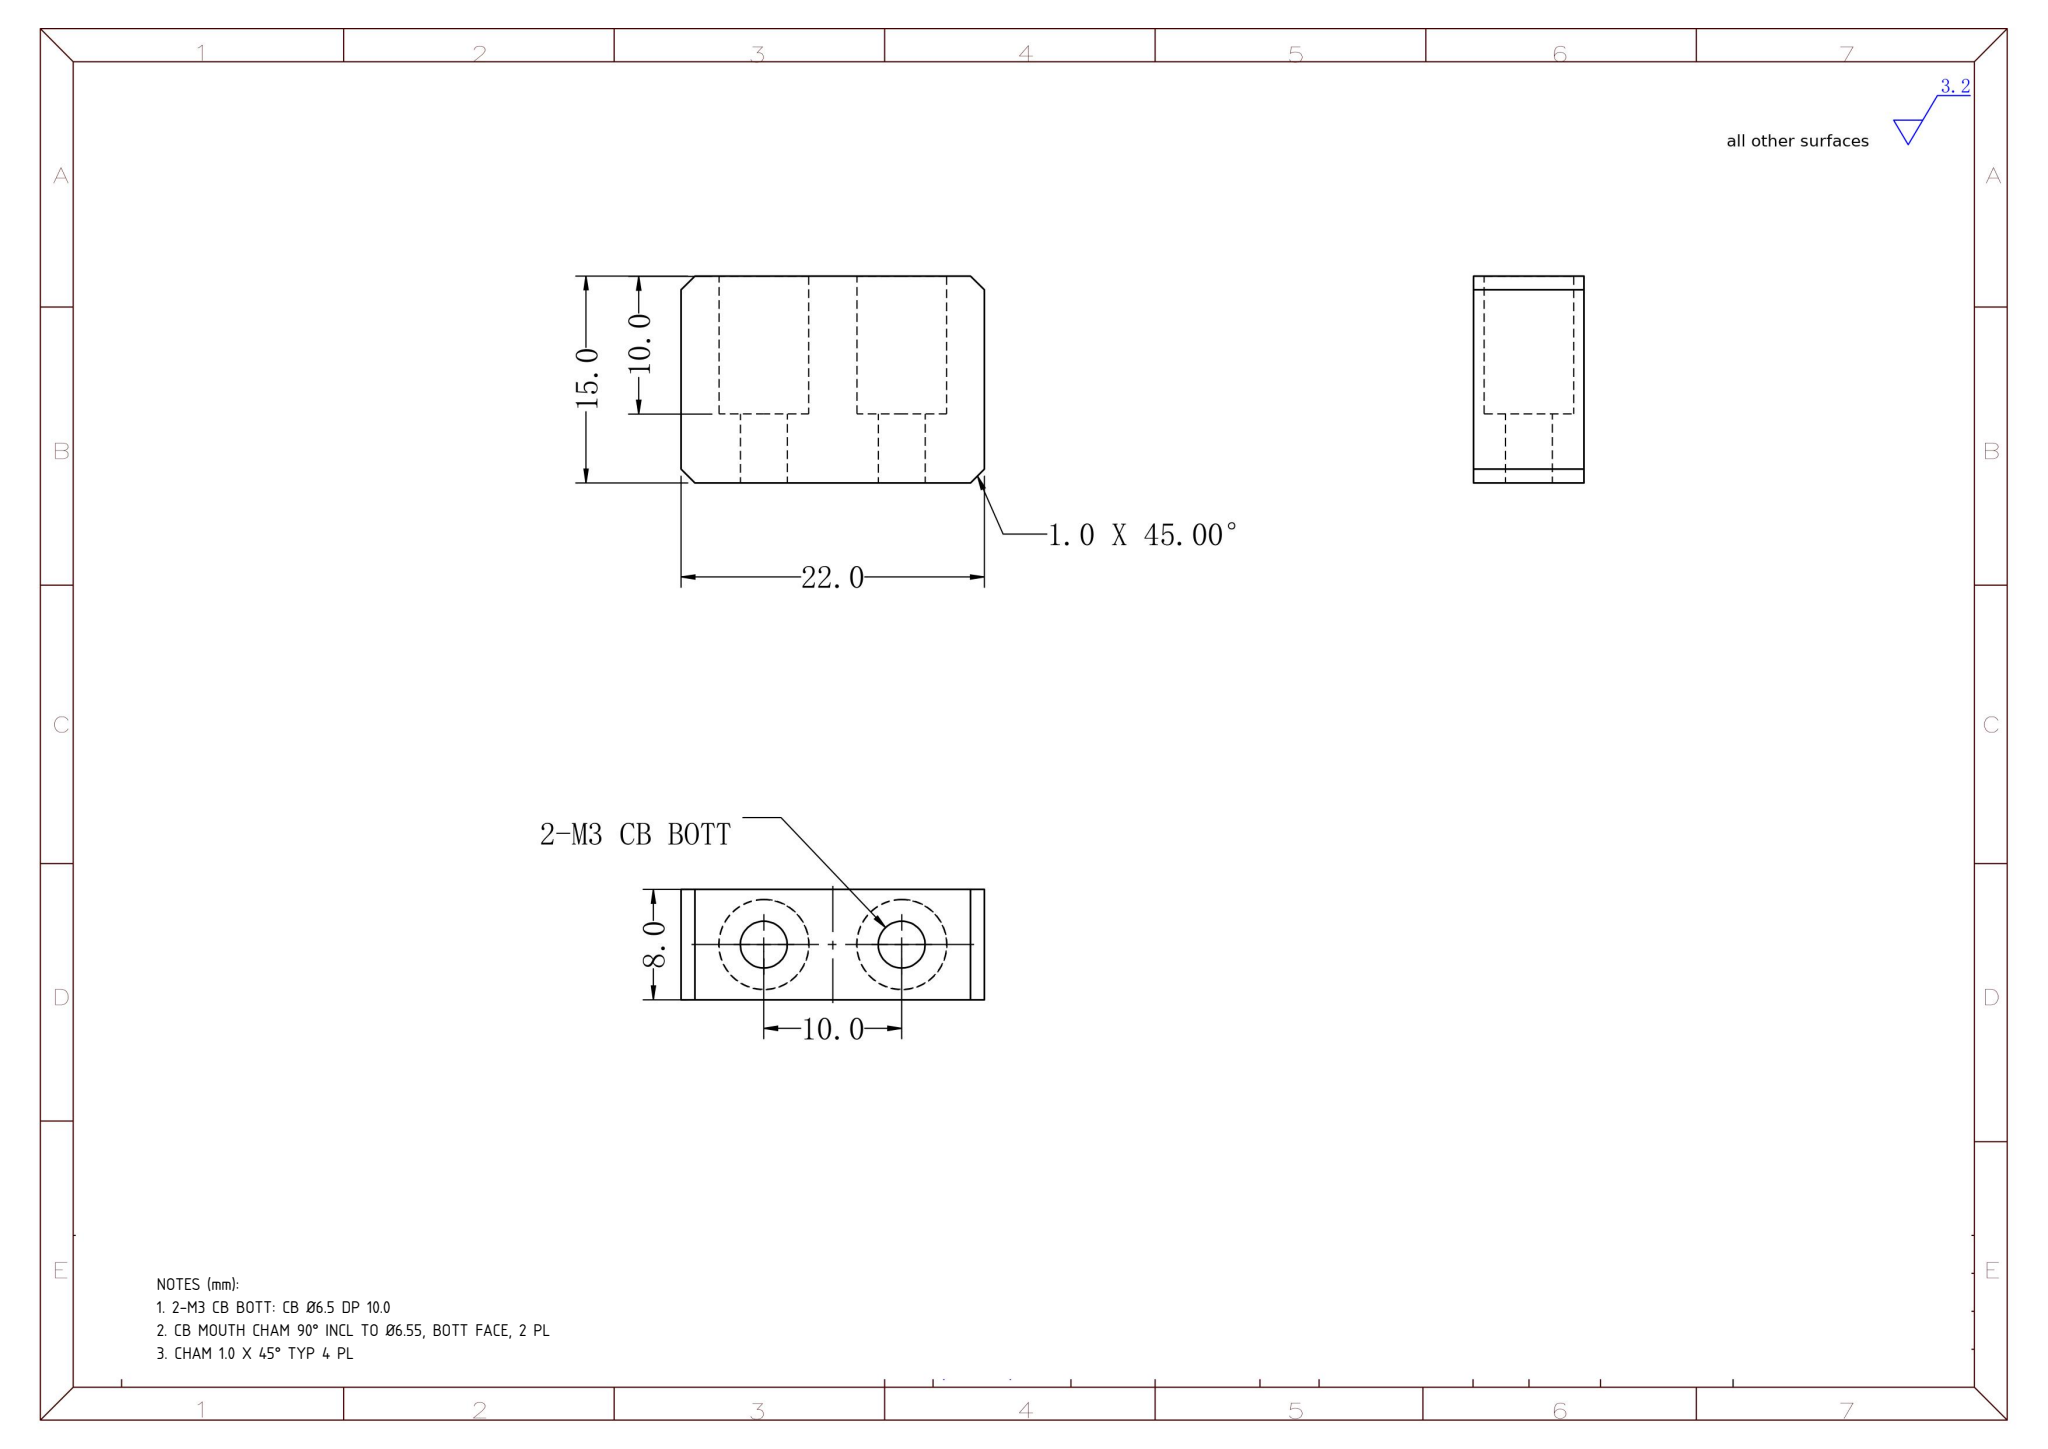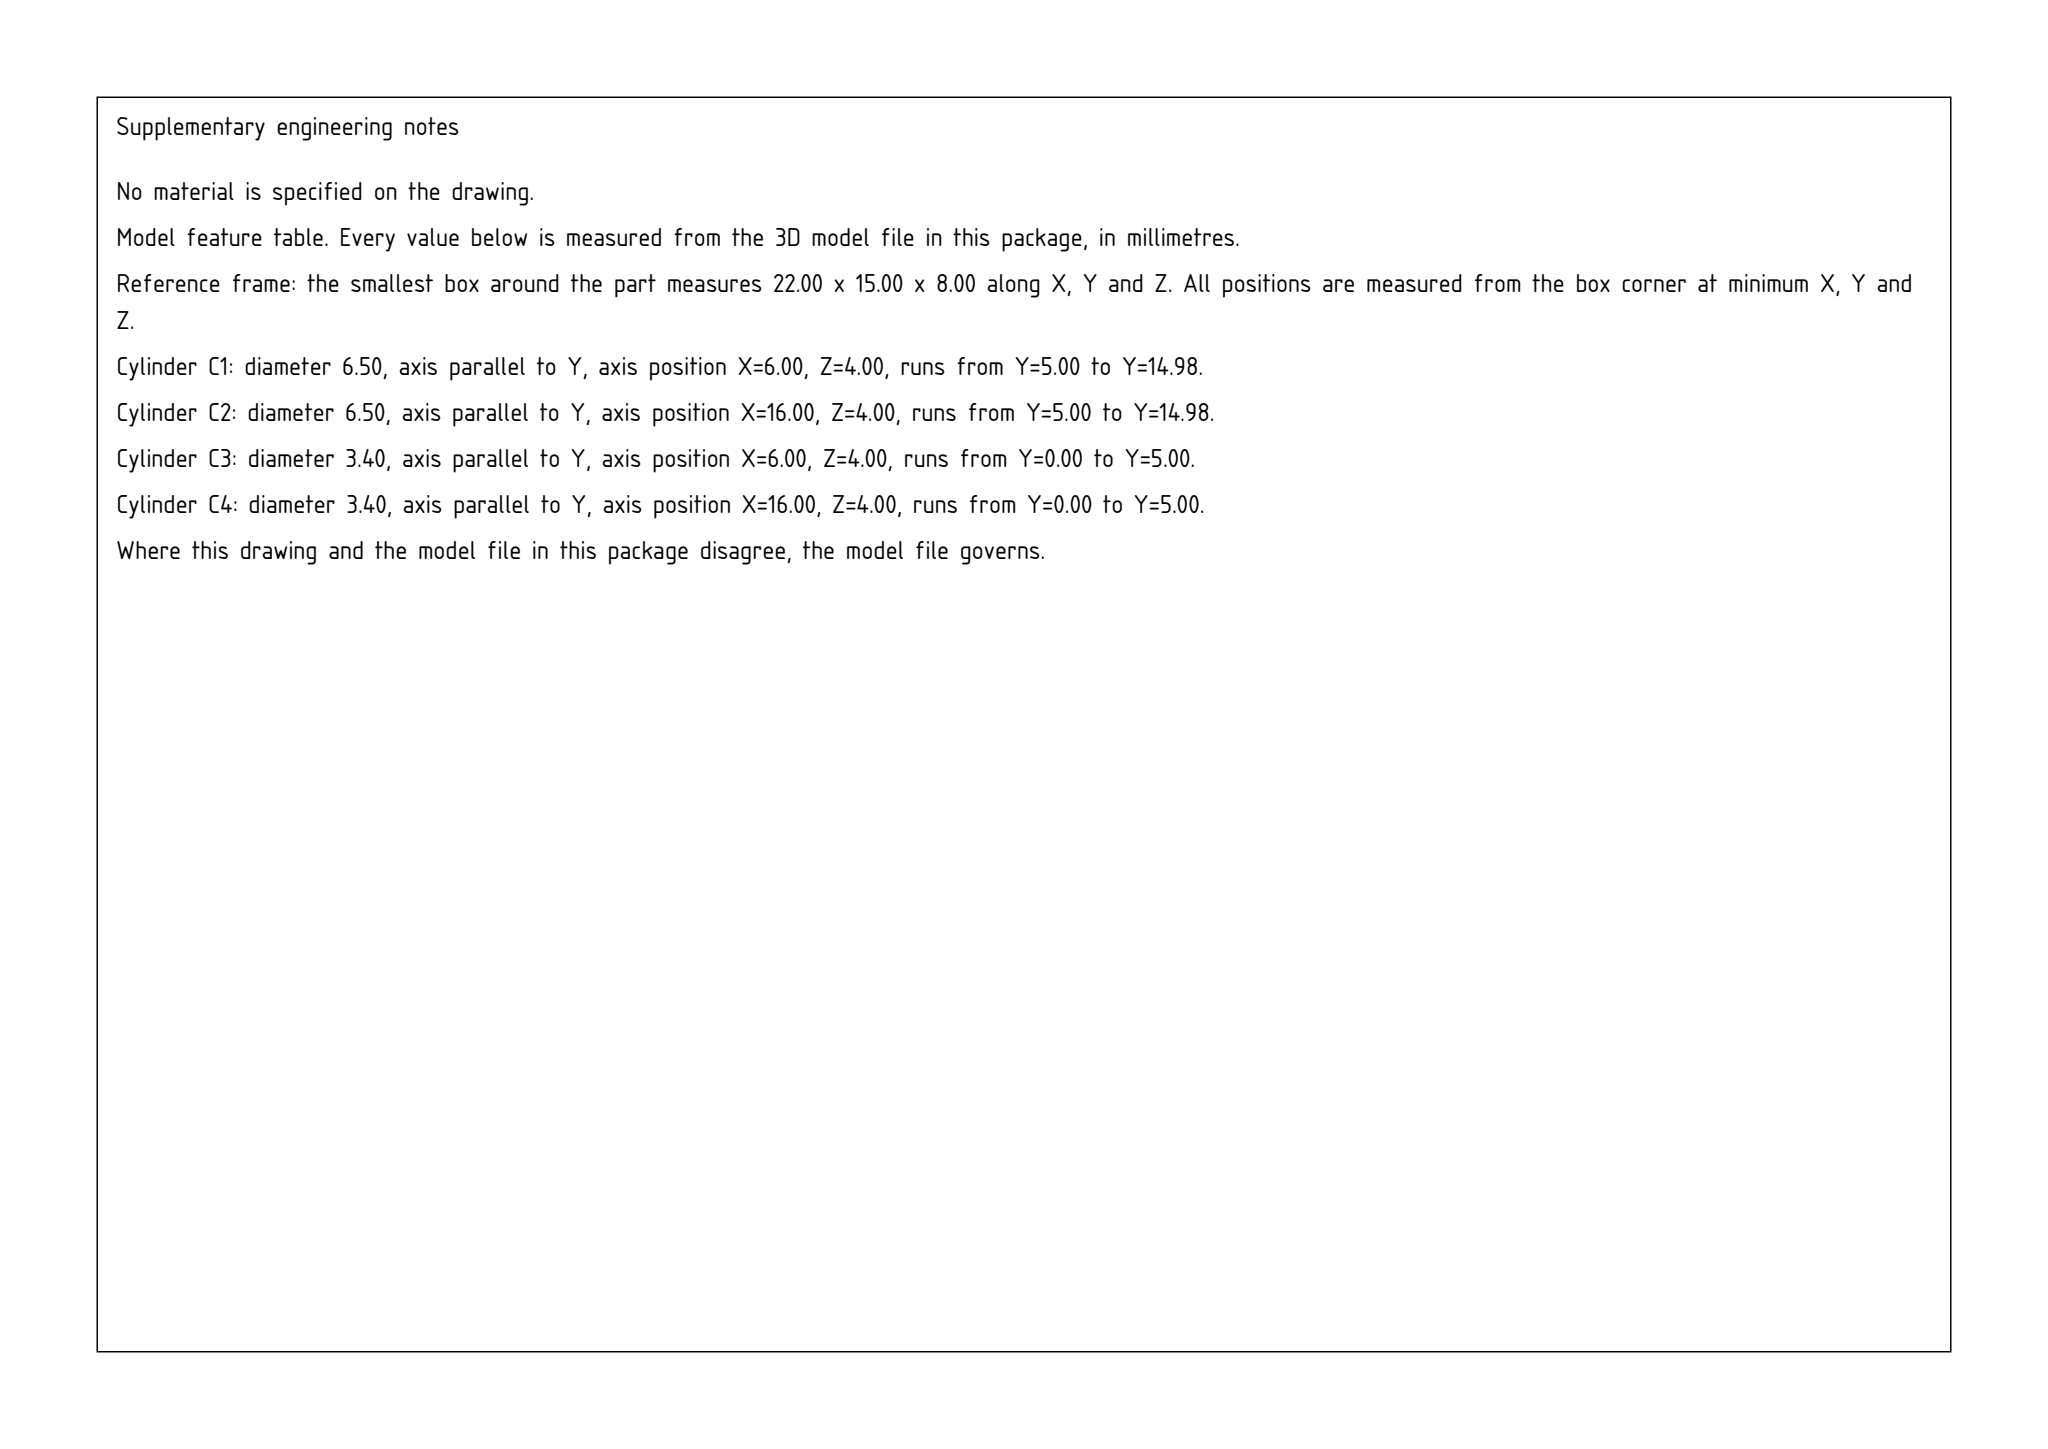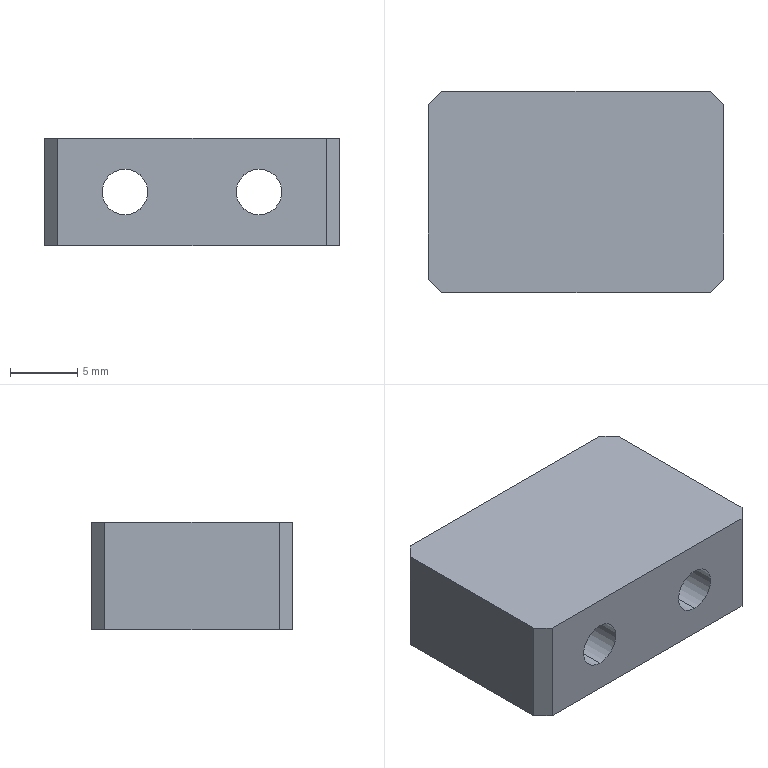Part | SolidWorks | mm | 1 solid | 24 faces | box 22 x 15 x 8 mm | volume 1870 mm3 | plane 12 | cylinder 8 | cone 4 | commonest cylinder face diameters 6.5 x4 3.4 x4
Drawing notes:
2-M3 CB BOTT: CB Ø6.5 DP 10.0 | from the solid: cylinders dia 6.5, axis y, at x=6.0 & 16.0, z=4.0, length 9.98 (y=5 to 15); matches 10.0 dim
CB MOUTH CHAM 90° INCL TO Ø6.55, BOTT FACE, 2 PL | from the solid: cones[included_angle 90.0, ref_dia 6.55] at Ø6.5 CB ends
CHAM 1.0 X 45° TYP 4 PL | from the solid: 4 corner chamfers on 22.0 x 15.0 outline, x-planes 0/22, y-planes 0/15
build123d program:
from build123d import *

# Parameters (mm, degrees)
SKETCH1_W                                      = 22
SKETCH1_H                                      = 15
BOSS_EXTRUDE1_DEPTH                            = 8
CHAMFER1_SIZE                                  = 1
M3_HEX_SOCKET_HEAD_CAP_SCREW_CBORE1_AT_2_COUNT = 2
M3_HEX_SOCKET_HEAD_CAP_SCREW_CBORE1_AT_2_PITCH = 10


with BuildPart() as part:
    # Sketch1 → Boss-Extrude1 (new body)
    with BuildSketch(Plane.XY):
        Rectangle(SKETCH1_W, SKETCH1_H)
    extrude(amount=BOSS_EXTRUDE1_DEPTH)

    # Chamfer1
    chamfer1_edges = [part.edges().sort_by_distance(p)[0] for p in [
        (11, -7.5, 4),
        (-11, -7.5, 4),
        (-11, 7.5, 4),
        (11, 7.5, 4),
    ]]
    chamfer(chamfer1_edges, length=CHAMFER1_SIZE)

    # Sketch7 → M3 Hex Socket Head Cap Screw CBORE1 (revolve, cut)
    with BuildSketch(Plane(origin=(-5, 7.5, 4), x_dir=(0, 0, 1), z_dir=(1, 0, 0))):
        Polygon((0, 0), (0, 15), (1.7, 15), (1.7, 10), (3.25, 10), (3.25, 0.025), (3.275, 0), align=None)
    m3_hex_socket_head_cap_screw_cbore1 = revolve(axis=Axis((-5, 13.85, 4), (0, -1, 0)), mode=Mode.SUBTRACT)

    # M3 Hex Socket Head Cap Screw CBORE1 at 2: M3 Hex Socket Head Cap Screw CBORE1 ×2
    with Locations(*[(i * M3_HEX_SOCKET_HEAD_CAP_SCREW_CBORE1_AT_2_PITCH, 0, 0) for i in range(1, M3_HEX_SOCKET_HEAD_CAP_SCREW_CBORE1_AT_2_COUNT)]):
        add(m3_hex_socket_head_cap_screw_cbore1, mode=Mode.SUBTRACT)


solid = part.part
STEP:
#1=CARTESIAN_POINT('',(-5.,7.475,0.75));
#2=VERTEX_POINT('',#1);
#3=CARTESIAN_POINT('',(-5.,7.475,7.25));
#4=VERTEX_POINT('',#3);
#5=CARTESIAN_POINT('',(-5.,7.475,4.));
#6=DIRECTION('',(0.,1.,0.));
#7=DIRECTION('',(0.,0.,1.));
#8=AXIS2_PLACEMENT_3D('',#5,#6,#7);
#9=CIRCLE('',#8,3.25);
#10=EDGE_CURVE('',#2,#4,#9,.T.);
#11=ORIENTED_EDGE('',*,*,#10,.F.);
#12=CARTESIAN_POINT('',(-5.,7.5,0.725));
#13=VERTEX_POINT('',#12);
#14=CARTESIAN_POINT('',(-5.,7.5,0.725));
#15=DIRECTION('',(0.,0.7071,-0.7071));
#16=VECTOR('',#15,1000.);
#17=LINE('',#14,#16);
#18=EDGE_CURVE('',#2,#13,#17,.T.);
#19=ORIENTED_EDGE('',*,*,#18,.T.);
#20=CARTESIAN_POINT('',(-5.,7.5,7.275));
#21=VERTEX_POINT('',#20);
#22=CARTESIAN_POINT('',(-5.,7.5,4.));
#23=DIRECTION('',(0.,1.,0.));
#24=DIRECTION('',(0.,0.,1.));
#25=AXIS2_PLACEMENT_3D('',#22,#23,#24);
#26=CIRCLE('',#25,3.275);
#27=EDGE_CURVE('',#13,#21,#26,.T.);
#28=ORIENTED_EDGE('',*,*,#27,.T.);
#29=CARTESIAN_POINT('',(-5.,7.5,7.275));
#30=DIRECTION('',(0.,0.7071,0.7071));
#31=VECTOR('',#30,1000.);
#32=LINE('',#29,#31);
#33=EDGE_CURVE('',#4,#21,#32,.T.);
#34=ORIENTED_EDGE('',*,*,#33,.F.);
#35=EDGE_LOOP('',(#11,#19,#28,#34));
#36=FACE_OUTER_BOUND('',#35,.T.);
#37=CARTESIAN_POINT('',(-5.,7.5,4.));
#38=DIRECTION('',(0.,1.,0.));
#39=DIRECTION('',(0.,0.,1.));
#40=AXIS2_PLACEMENT_3D('',#37,#38,#39);
#41=CONICAL_SURFACE('',#40,3.275,0.7854);
#42=ADVANCED_FACE('',(#36),#41,.F.);
#43=CARTESIAN_POINT('',(-5.,-2.5,0.75));
#44=VERTEX_POINT('',#43);
#45=CARTESIAN_POINT('',(-5.,-2.5,7.25));
#46=VERTEX_POINT('',#45);
#47=CARTESIAN_POINT('',(-5.,-2.5,4.));
#48=DIRECTION('',(0.,1.,0.));
#49=DIRECTION('',(0.,0.,1.));
#50=AXIS2_PLACEMENT_3D('',#47,#48,#49);
#51=CIRCLE('',#50,3.25);
#52=EDGE_CURVE('',#44,#46,#51,.T.);
#53=ORIENTED_EDGE('',*,*,#52,.F.);
#54=CARTESIAN_POINT('',(-5.,7.5,0.75));
#55=DIRECTION('',(0.,1.,0.));
#56=VECTOR('',#55,1000.);
#57=LINE('',#54,#56);
#58=EDGE_CURVE('',#44,#2,#57,.T.);
#59=ORIENTED_EDGE('',*,*,#58,.T.);
#60=ORIENTED_EDGE('',*,*,#10,.T.);
#61=CARTESIAN_POINT('',(-5.,7.5,7.25));
#62=DIRECTION('',(0.,1.,0.));
#63=VECTOR('',#62,1000.);
#64=LINE('',#61,#63);
#65=EDGE_CURVE('',#46,#4,#64,.T.);
#66=ORIENTED_EDGE('',*,*,#65,.F.);
#67=EDGE_LOOP('',(#53,#59,#60,#66));
#68=FACE_OUTER_BOUND('',#67,.T.);
#69=CARTESIAN_POINT('',(-5.,7.5,4.));
#70=DIRECTION('',(0.,1.,0.));
#71=DIRECTION('',(0.,0.,1.));
#72=AXIS2_PLACEMENT_3D('',#69,#70,#71);
#73=CYLINDRICAL_SURFACE('',#72,3.25);
#74=ADVANCED_FACE('',(#68),#73,.F.);
#75=CARTESIAN_POINT('',(-5.,-7.5,2.3));
#76=VERTEX_POINT('',#75);
#77=CARTESIAN_POINT('',(-5.,-7.5,5.7));
#78=VERTEX_POINT('',#77);
#79=CARTESIAN_POINT('',(-5.,-7.5,4.));
#80=DIRECTION('',(0.,1.,0.));
#81=DIRECTION('',(0.,0.,1.));
#82=AXIS2_PLACEMENT_3D('',#79,#80,#81);
#83=CIRCLE('',#82,1.7);
#84=EDGE_CURVE('',#76,#78,#83,.T.);
#85=ORIENTED_EDGE('',*,*,#84,.F.);
#86=CARTESIAN_POINT('',(-5.,-2.5,2.3));
#87=VERTEX_POINT('',#86);
#88=CARTESIAN_POINT('',(-5.,7.5,2.3));
#89=DIRECTION('',(0.,1.,0.));
#90=VECTOR('',#89,1000.);
#91=LINE('',#88,#90);
#92=EDGE_CURVE('',#76,#87,#91,.T.);
#93=ORIENTED_EDGE('',*,*,#92,.T.);
#94=CARTESIAN_POINT('',(-5.,-2.5,5.7));
#95=VERTEX_POINT('',#94);
#96=CARTESIAN_POINT('',(-5.,-2.5,4.));
#97=DIRECTION('',(0.,1.,0.));
#98=DIRECTION('',(0.,0.,1.));
#99=AXIS2_PLACEMENT_3D('',#96,#97,#98);
#100=CIRCLE('',#99,1.7);
#101=EDGE_CURVE('',#87,#95,#100,.T.);
#102=ORIENTED_EDGE('',*,*,#101,.T.);
#103=CARTESIAN_POINT('',(-5.,7.5,5.7));
#104=DIRECTION('',(0.,1.,0.));
#105=VECTOR('',#104,1000.);
#106=LINE('',#103,#105);
#107=EDGE_CURVE('',#78,#95,#106,.T.);
#108=ORIENTED_EDGE('',*,*,#107,.F.);
#109=EDGE_LOOP('',(#85,#93,#102,#108));
#110=FACE_OUTER_BOUND('',#109,.T.);
#111=CARTESIAN_POINT('',(-5.,7.5,4.));
#112=DIRECTION('',(0.,1.,0.));
#113=DIRECTION('',(0.,0.,1.));
#114=AXIS2_PLACEMENT_3D('',#111,#112,#113);
#115=CYLINDRICAL_SURFACE('',#114,1.7);
#116=ADVANCED_FACE('',(#110),#115,.F.);
#117=CARTESIAN_POINT('',(5.,7.475,0.75));
#118=VERTEX_POINT('',#117);
#119=CARTESIAN_POINT('',(5.,7.475,7.25));
#120=VERTEX_POINT('',#119);
#121=CARTESIAN_POINT('',(5.,7.475,4.));
#122=DIRECTION('',(0.,1.,0.));
#123=DIRECTION('',(0.,0.,1.));
#124=AXIS2_PLACEMENT_3D('',#121,#122,#123);
#125=CIRCLE('',#124,3.25);
#126=EDGE_CURVE('',#118,#120,#125,.T.);
#127=ORIENTED_EDGE('',*,*,#126,.F.);
#128=CARTESIAN_POINT('',(5.,7.5,0.725));
#129=VERTEX_POINT('',#128);
#130=CARTESIAN_POINT('',(5.,7.5,0.725));
#131=DIRECTION('',(0.,0.7071,-0.7071));
#132=VECTOR('',#131,1000.);
#133=LINE('',#130,#132);
#134=EDGE_CURVE('',#118,#129,#133,.T.);
#135=ORIENTED_EDGE('',*,*,#134,.T.);
#136=CARTESIAN_POINT('',(5.,7.5,7.275));
#137=VERTEX_POINT('',#136);
#138=CARTESIAN_POINT('',(5.,7.5,4.));
#139=DIRECTION('',(0.,1.,0.));
#140=DIRECTION('',(0.,0.,1.));
#141=AXIS2_PLACEMENT_3D('',#138,#139,#140);
#142=CIRCLE('',#141,3.275);
#143=EDGE_CURVE('',#129,#137,#142,.T.);
#144=ORIENTED_EDGE('',*,*,#143,.T.);
#145=CARTESIAN_POINT('',(5.,7.5,7.275));
#146=DIRECTION('',(0.,0.7071,0.7071));
#147=VECTOR('',#146,1000.);
#148=LINE('',#145,#147);
#149=EDGE_CURVE('',#120,#137,#148,.T.);
#150=ORIENTED_EDGE('',*,*,#149,.F.);
#151=EDGE_LOOP('',(#127,#135,#144,#150));
#152=FACE_OUTER_BOUND('',#151,.T.);
#153=CARTESIAN_POINT('',(5.,7.5,4.));
#154=DIRECTION('',(0.,1.,0.));
#155=DIRECTION('',(0.,0.,1.));
#156=AXIS2_PLACEMENT_3D('',#153,#154,#155);
#157=CONICAL_SURFACE('',#156,3.275,0.7854);
#158=ADVANCED_FACE('',(#152),#157,.F.);
#159=CARTESIAN_POINT('',(5.,-2.5,0.75));
#160=VERTEX_POINT('',#159);
#161=CARTESIAN_POINT('',(5.,-2.5,7.25));
#162=VERTEX_POINT('',#161);
#163=CARTESIAN_POINT('',(5.,-2.5,4.));
#164=DIRECTION('',(0.,1.,0.));
#165=DIRECTION('',(0.,0.,1.));
#166=AXIS2_PLACEMENT_3D('',#163,#164,#165);
#167=CIRCLE('',#166,3.25);
#168=EDGE_CURVE('',#160,#162,#167,.T.);
#169=ORIENTED_EDGE('',*,*,#168,.F.);
#170=CARTESIAN_POINT('',(5.,7.5,0.75));
#171=DIRECTION('',(0.,1.,0.));
#172=VECTOR('',#171,1000.);
#173=LINE('',#170,#172);
#174=EDGE_CURVE('',#160,#118,#173,.T.);
#175=ORIENTED_EDGE('',*,*,#174,.T.);
#176=ORIENTED_EDGE('',*,*,#126,.T.);
#177=CARTESIAN_POINT('',(5.,7.5,7.25));
#178=DIRECTION('',(0.,1.,0.));
#179=VECTOR('',#178,1000.);
#180=LINE('',#177,#179);
#181=EDGE_CURVE('',#162,#120,#180,.T.);
#182=ORIENTED_EDGE('',*,*,#181,.F.);
#183=EDGE_LOOP('',(#169,#175,#176,#182));
#184=FACE_OUTER_BOUND('',#183,.T.);
#185=CARTESIAN_POINT('',(5.,7.5,4.));
#186=DIRECTION('',(0.,1.,0.));
#187=DIRECTION('',(0.,0.,1.));
#188=AXIS2_PLACEMENT_3D('',#185,#186,#187);
#189=CYLINDRICAL_SURFACE('',#188,3.25);
#190=ADVANCED_FACE('',(#184),#189,.F.);
#191=CARTESIAN_POINT('',(5.,-7.5,2.3));
#192=VERTEX_POINT('',#191);
#193=CARTESIAN_POINT('',(5.,-7.5,5.7));
#194=VERTEX_POINT('',#193);
#195=CARTESIAN_POINT('',(5.,-7.5,4.));
#196=DIRECTION('',(0.,1.,0.));
#197=DIRECTION('',(0.,0.,1.));
#198=AXIS2_PLACEMENT_3D('',#195,#196,#197);
#199=CIRCLE('',#198,1.7);
#200=EDGE_CURVE('',#192,#194,#199,.T.);
#201=ORIENTED_EDGE('',*,*,#200,.F.);
#202=CARTESIAN_POINT('',(5.,-2.5,2.3));
#203=VERTEX_POINT('',#202);
#204=CARTESIAN_POINT('',(5.,7.5,2.3));
#205=DIRECTION('',(0.,1.,0.));
#206=VECTOR('',#205,1000.);
#207=LINE('',#204,#206);
#208=EDGE_CURVE('',#192,#203,#207,.T.);
#209=ORIENTED_EDGE('',*,*,#208,.T.);
#210=CARTESIAN_POINT('',(5.,-2.5,5.7));
#211=VERTEX_POINT('',#210);
#212=CARTESIAN_POINT('',(5.,-2.5,4.));
#213=DIRECTION('',(0.,1.,0.));
#214=DIRECTION('',(0.,0.,1.));
#215=AXIS2_PLACEMENT_3D('',#212,#213,#214);
#216=CIRCLE('',#215,1.7);
#217=EDGE_CURVE('',#203,#211,#216,.T.);
#218=ORIENTED_EDGE('',*,*,#217,.T.);
#219=CARTESIAN_POINT('',(5.,7.5,5.7));
#220=DIRECTION('',(0.,1.,0.));
#221=VECTOR('',#220,1000.);
#222=LINE('',#219,#221);
#223=EDGE_CURVE('',#194,#211,#222,.T.);
#224=ORIENTED_EDGE('',*,*,#223,.F.);
#225=EDGE_LOOP('',(#201,#209,#218,#224));
#226=FACE_OUTER_BOUND('',#225,.T.);
#227=CARTESIAN_POINT('',(5.,7.5,4.));
#228=DIRECTION('',(0.,1.,0.));
#229=DIRECTION('',(0.,0.,1.));
#230=AXIS2_PLACEMENT_3D('',#227,#228,#229);
#231=CYLINDRICAL_SURFACE('',#230,1.7);
#232=ADVANCED_FACE('',(#226),#231,.F.);
#233=CARTESIAN_POINT('',(11.,-6.5,8.));
#234=VERTEX_POINT('',#233);
#235=CARTESIAN_POINT('',(11.,6.5,8.));
#236=VERTEX_POINT('',#235);
#237=CARTESIAN_POINT('',(11.,7.5,8.));
#238=DIRECTION('',(-0.,1.,0.));
#239=VECTOR('',#238,1000.);
#240=LINE('',#237,#239);
#241=EDGE_CURVE('',#234,#236,#240,.T.);
#242=ORIENTED_EDGE('',*,*,#241,.F.);
#243=CARTESIAN_POINT('',(11.,-6.5,0.));
#244=VERTEX_POINT('',#243);
#245=CARTESIAN_POINT('',(11.,-6.5,8.));
#246=DIRECTION('',(0.,0.,-1.));
#247=VECTOR('',#246,1000.);
#248=LINE('',#245,#247);
#249=EDGE_CURVE('',#234,#244,#248,.T.);
#250=ORIENTED_EDGE('',*,*,#249,.T.);
#251=CARTESIAN_POINT('',(11.,6.5,0.));
#252=VERTEX_POINT('',#251);
#253=CARTESIAN_POINT('',(11.,7.5,0.));
#254=DIRECTION('',(-0.,1.,0.));
#255=VECTOR('',#254,1000.);
#256=LINE('',#253,#255);
#257=EDGE_CURVE('',#244,#252,#256,.T.);
#258=ORIENTED_EDGE('',*,*,#257,.T.);
#259=CARTESIAN_POINT('',(11.,6.5,8.));
#260=DIRECTION('',(0.,0.,1.));
#261=VECTOR('',#260,1000.);
#262=LINE('',#259,#261);
#263=EDGE_CURVE('',#252,#236,#262,.T.);
#264=ORIENTED_EDGE('',*,*,#263,.T.);
#265=EDGE_LOOP('',(#242,#250,#258,#264));
#266=FACE_OUTER_BOUND('',#265,.T.);
#267=CARTESIAN_POINT('',(11.,7.5,8.));
#268=DIRECTION('',(-1.,-0.,0.));
#269=DIRECTION('',(0.,-1.,0.));
#270=AXIS2_PLACEMENT_3D('',#267,#268,#269);
#271=PLANE('',#270);
#272=ADVANCED_FACE('',(#266),#271,.F.);
#273=CARTESIAN_POINT('',(-5.,7.5,4.));
#274=DIRECTION('',(0.,1.,0.));
#275=DIRECTION('',(0.,0.,1.));
#276=AXIS2_PLACEMENT_3D('',#273,#274,#275);
#277=CIRCLE('',#276,3.275);
#278=EDGE_CURVE('',#21,#13,#277,.T.);
#279=ORIENTED_EDGE('',*,*,#278,.F.);
#280=ORIENTED_EDGE('',*,*,#27,.F.);
#281=EDGE_LOOP('',(#279,#280));
#282=FACE_BOUND('',#281,.T.);
#283=CARTESIAN_POINT('',(5.,7.5,4.));
#284=DIRECTION('',(0.,1.,0.));
#285=DIRECTION('',(0.,0.,1.));
#286=AXIS2_PLACEMENT_3D('',#283,#284,#285);
#287=CIRCLE('',#286,3.275);
#288=EDGE_CURVE('',#137,#129,#287,.T.);
#289=ORIENTED_EDGE('',*,*,#288,.F.);
#290=ORIENTED_EDGE('',*,*,#143,.F.);
#291=EDGE_LOOP('',(#289,#290));
#292=FACE_BOUND('',#291,.T.);
#293=CARTESIAN_POINT('',(10.,7.5,8.));
#294=VERTEX_POINT('',#293);
#295=CARTESIAN_POINT('',(-10.,7.5,8.));
#296=VERTEX_POINT('',#295);
#297=CARTESIAN_POINT('',(-11.,7.5,8.));
#298=DIRECTION('',(-1.,0.,0.));
#299=VECTOR('',#298,1000.);
#300=LINE('',#297,#299);
#301=EDGE_CURVE('',#294,#296,#300,.T.);
#302=ORIENTED_EDGE('',*,*,#301,.F.);
#303=CARTESIAN_POINT('',(10.,7.5,0.));
#304=VERTEX_POINT('',#303);
#305=CARTESIAN_POINT('',(10.,7.5,8.));
#306=DIRECTION('',(0.,0.,-1.));
#307=VECTOR('',#306,1000.);
#308=LINE('',#305,#307);
#309=EDGE_CURVE('',#294,#304,#308,.T.);
#310=ORIENTED_EDGE('',*,*,#309,.T.);
#311=CARTESIAN_POINT('',(-10.,7.5,0.));
#312=VERTEX_POINT('',#311);
#313=CARTESIAN_POINT('',(-11.,7.5,0.));
#314=DIRECTION('',(-1.,0.,0.));
#315=VECTOR('',#314,1000.);
#316=LINE('',#313,#315);
#317=EDGE_CURVE('',#304,#312,#316,.T.);
#318=ORIENTED_EDGE('',*,*,#317,.T.);
#319=CARTESIAN_POINT('',(-10.,7.5,8.));
#320=DIRECTION('',(0.,0.,1.));
#321=VECTOR('',#320,1000.);
#322=LINE('',#319,#321);
#323=EDGE_CURVE('',#312,#296,#322,.T.);
#324=ORIENTED_EDGE('',*,*,#323,.T.);
#325=EDGE_LOOP('',(#302,#310,#318,#324));
#326=FACE_OUTER_BOUND('',#325,.T.);
#327=CARTESIAN_POINT('',(-11.,7.5,8.));
#328=DIRECTION('',(0.,-1.,0.));
#329=DIRECTION('',(0.,0.,-1.));
#330=AXIS2_PLACEMENT_3D('',#327,#328,#329);
#331=PLANE('',#330);
#332=ADVANCED_FACE('',(#282,#292,#326),#331,.F.);
#333=CARTESIAN_POINT('',(-11.,6.5,0.));
#334=VERTEX_POINT('',#333);
#335=CARTESIAN_POINT('',(-11.,-6.5,0.));
#336=VERTEX_POINT('',#335);
#337=CARTESIAN_POINT('',(-11.,7.5,0.));
#338=DIRECTION('',(0.,-1.,0.));
#339=VECTOR('',#338,1000.);
#340=LINE('',#337,#339);
#341=EDGE_CURVE('',#334,#336,#340,.T.);
#342=ORIENTED_EDGE('',*,*,#341,.T.);
#343=CARTESIAN_POINT('',(-11.,-6.5,8.));
#344=VERTEX_POINT('',#343);
#345=CARTESIAN_POINT('',(-11.,-6.5,8.));
#346=DIRECTION('',(0.,0.,1.));
#347=VECTOR('',#346,1000.);
#348=LINE('',#345,#347);
#349=EDGE_CURVE('',#336,#344,#348,.T.);
#350=ORIENTED_EDGE('',*,*,#349,.T.);
#351=CARTESIAN_POINT('',(-11.,6.5,8.));
#352=VERTEX_POINT('',#351);
#353=CARTESIAN_POINT('',(-11.,7.5,8.));
#354=DIRECTION('',(0.,-1.,0.));
#355=VECTOR('',#354,1000.);
#356=LINE('',#353,#355);
#357=EDGE_CURVE('',#352,#344,#356,.T.);
#358=ORIENTED_EDGE('',*,*,#357,.F.);
#359=CARTESIAN_POINT('',(-11.,6.5,8.));
#360=DIRECTION('',(0.,0.,-1.));
#361=VECTOR('',#360,1000.);
#362=LINE('',#359,#361);
#363=EDGE_CURVE('',#352,#334,#362,.T.);
#364=ORIENTED_EDGE('',*,*,#363,.T.);
#365=EDGE_LOOP('',(#342,#350,#358,#364));
#366=FACE_OUTER_BOUND('',#365,.T.);
#367=CARTESIAN_POINT('',(-11.,7.5,8.));
#368=DIRECTION('',(1.,0.,0.));
#369=DIRECTION('',(-0.,1.,0.));
#370=AXIS2_PLACEMENT_3D('',#367,#368,#369);
#371=PLANE('',#370);
#372=ADVANCED_FACE('',(#366),#371,.F.);
#373=CARTESIAN_POINT('',(-5.,-7.5,4.));
#374=DIRECTION('',(0.,1.,0.));
#375=DIRECTION('',(0.,0.,1.));
#376=AXIS2_PLACEMENT_3D('',#373,#374,#375);
#377=CIRCLE('',#376,1.7);
#378=EDGE_CURVE('',#78,#76,#377,.T.);
#379=ORIENTED_EDGE('',*,*,#378,.T.);
#380=ORIENTED_EDGE('',*,*,#84,.T.);
#381=EDGE_LOOP('',(#379,#380));
#382=FACE_BOUND('',#381,.T.);
#383=CARTESIAN_POINT('',(5.,-7.5,4.));
#384=DIRECTION('',(0.,1.,0.));
#385=DIRECTION('',(0.,0.,1.));
#386=AXIS2_PLACEMENT_3D('',#383,#384,#385);
#387=CIRCLE('',#386,1.7);
#388=EDGE_CURVE('',#194,#192,#387,.T.);
#389=ORIENTED_EDGE('',*,*,#388,.T.);
#390=ORIENTED_EDGE('',*,*,#200,.T.);
#391=EDGE_LOOP('',(#389,#390));
#392=FACE_BOUND('',#391,.T.);
#393=CARTESIAN_POINT('',(-10.,-7.5,0.));
#394=VERTEX_POINT('',#393);
#395=CARTESIAN_POINT('',(10.,-7.5,0.));
#396=VERTEX_POINT('',#395);
#397=CARTESIAN_POINT('',(-11.,-7.5,0.));
#398=DIRECTION('',(1.,0.,0.));
#399=VECTOR('',#398,1000.);
#400=LINE('',#397,#399);
#401=EDGE_CURVE('',#394,#396,#400,.T.);
#402=ORIENTED_EDGE('',*,*,#401,.T.);
#403=CARTESIAN_POINT('',(10.,-7.5,8.));
#404=VERTEX_POINT('',#403);
#405=CARTESIAN_POINT('',(10.,-7.5,8.));
#406=DIRECTION('',(0.,0.,1.));
#407=VECTOR('',#406,1000.);
#408=LINE('',#405,#407);
#409=EDGE_CURVE('',#396,#404,#408,.T.);
#410=ORIENTED_EDGE('',*,*,#409,.T.);
#411=CARTESIAN_POINT('',(-10.,-7.5,8.));
#412=VERTEX_POINT('',#411);
#413=CARTESIAN_POINT('',(-11.,-7.5,8.));
#414=DIRECTION('',(1.,0.,0.));
#415=VECTOR('',#414,1000.);
#416=LINE('',#413,#415);
#417=EDGE_CURVE('',#412,#404,#416,.T.);
#418=ORIENTED_EDGE('',*,*,#417,.F.);
#419=CARTESIAN_POINT('',(-10.,-7.5,8.));
#420=DIRECTION('',(0.,0.,-1.));
#421=VECTOR('',#420,1000.);
#422=LINE('',#419,#421);
#423=EDGE_CURVE('',#412,#394,#422,.T.);
#424=ORIENTED_EDGE('',*,*,#423,.T.);
#425=EDGE_LOOP('',(#402,#410,#418,#424));
#426=FACE_OUTER_BOUND('',#425,.T.);
#427=CARTESIAN_POINT('',(-11.,-7.5,8.));
#428=DIRECTION('',(0.,1.,0.));
#429=DIRECTION('',(0.,0.,1.));
#430=AXIS2_PLACEMENT_3D('',#427,#428,#429);
#431=PLANE('',#430);
#432=ADVANCED_FACE('',(#382,#392,#426),#431,.F.);
#433=ORIENTED_EDGE('',*,*,#417,.T.);
#434=CARTESIAN_POINT('',(8.75,-8.75,8.));
#435=DIRECTION('',(0.7071,0.7071,0.));
#436=VECTOR('',#435,1000.);
#437=LINE('',#434,#436);
#438=EDGE_CURVE('',#404,#234,#437,.T.);
#439=ORIENTED_EDGE('',*,*,#438,.T.);
#440=ORIENTED_EDGE('',*,*,#241,.T.);
#441=CARTESIAN_POINT('',(8.75,8.75,8.));
#442=DIRECTION('',(-0.7071,0.7071,0.));
#443=VECTOR('',#442,1000.);
#444=LINE('',#441,#443);
#445=EDGE_CURVE('',#236,#294,#444,.T.);
#446=ORIENTED_EDGE('',*,*,#445,.T.);
#447=ORIENTED_EDGE('',*,*,#301,.T.);
#448=CARTESIAN_POINT('',(-8.75,8.75,8.));
#449=DIRECTION('',(-0.7071,-0.7071,0.));
#450=VECTOR('',#449,1000.);
#451=LINE('',#448,#450);
#452=EDGE_CURVE('',#296,#352,#451,.T.);
#453=ORIENTED_EDGE('',*,*,#452,.T.);
#454=ORIENTED_EDGE('',*,*,#357,.T.);
#455=CARTESIAN_POINT('',(-8.75,-8.75,8.));
#456=DIRECTION('',(0.7071,-0.7071,0.));
#457=VECTOR('',#456,1000.);
#458=LINE('',#455,#457);
#459=EDGE_CURVE('',#344,#412,#458,.T.);
#460=ORIENTED_EDGE('',*,*,#459,.T.);
#461=EDGE_LOOP('',(#433,#439,#440,#446,#447,#453,#454,#460));
#462=FACE_OUTER_BOUND('',#461,.T.);
#463=CARTESIAN_POINT('',(0.,0.,8.));
#464=DIRECTION('',(0.,0.,1.));
#465=DIRECTION('',(1.,0.,0.));
#466=AXIS2_PLACEMENT_3D('',#463,#464,#465);
#467=PLANE('',#466);
#468=ADVANCED_FACE('',(#462),#467,.T.);
#469=ORIENTED_EDGE('',*,*,#257,.F.);
#470=CARTESIAN_POINT('',(11.,-6.5,0.));
#471=DIRECTION('',(-0.7071,-0.7071,0.));
#472=VECTOR('',#471,1000.);
#473=LINE('',#470,#472);
#474=EDGE_CURVE('',#244,#396,#473,.T.);
#475=ORIENTED_EDGE('',*,*,#474,.T.);
#476=ORIENTED_EDGE('',*,*,#401,.F.);
#477=CARTESIAN_POINT('',(-10.,-7.5,0.));
#478=DIRECTION('',(-0.7071,0.7071,0.));
#479=VECTOR('',#478,1000.);
#480=LINE('',#477,#479);
#481=EDGE_CURVE('',#394,#336,#480,.T.);
#482=ORIENTED_EDGE('',*,*,#481,.T.);
#483=ORIENTED_EDGE('',*,*,#341,.F.);
#484=CARTESIAN_POINT('',(-11.,6.5,0.));
#485=DIRECTION('',(0.7071,0.7071,0.));
#486=VECTOR('',#485,1000.);
#487=LINE('',#484,#486);
#488=EDGE_CURVE('',#334,#312,#487,.T.);
#489=ORIENTED_EDGE('',*,*,#488,.T.);
#490=ORIENTED_EDGE('',*,*,#317,.F.);
#491=CARTESIAN_POINT('',(10.,7.5,0.));
#492=DIRECTION('',(0.7071,-0.7071,0.));
#493=VECTOR('',#492,1000.);
#494=LINE('',#491,#493);
#495=EDGE_CURVE('',#304,#252,#494,.T.);
#496=ORIENTED_EDGE('',*,*,#495,.T.);
#497=EDGE_LOOP('',(#469,#475,#476,#482,#483,#489,#490,#496));
#498=FACE_OUTER_BOUND('',#497,.T.);
#499=CARTESIAN_POINT('',(0.,0.,0.));
#500=DIRECTION('',(0.,0.,1.));
#501=DIRECTION('',(1.,0.,0.));
#502=AXIS2_PLACEMENT_3D('',#499,#500,#501);
#503=PLANE('',#502);
#504=ADVANCED_FACE('',(#498),#503,.F.);
#505=ORIENTED_EDGE('',*,*,#438,.F.);
#506=ORIENTED_EDGE('',*,*,#409,.F.);
#507=ORIENTED_EDGE('',*,*,#474,.F.);
#508=ORIENTED_EDGE('',*,*,#249,.F.);
#509=EDGE_LOOP('',(#505,#506,#507,#508));
#510=FACE_OUTER_BOUND('',#509,.T.);
#511=CARTESIAN_POINT('',(11.,-6.5,8.));
#512=DIRECTION('',(-0.7071,0.7071,0.));
#513=DIRECTION('',(0.,0.,-1.));
#514=AXIS2_PLACEMENT_3D('',#511,#512,#513);
#515=PLANE('',#514);
#516=ADVANCED_FACE('',(#510),#515,.F.);
#517=ORIENTED_EDGE('',*,*,#445,.F.);
#518=ORIENTED_EDGE('',*,*,#263,.F.);
#519=ORIENTED_EDGE('',*,*,#495,.F.);
#520=ORIENTED_EDGE('',*,*,#309,.F.);
#521=EDGE_LOOP('',(#517,#518,#519,#520));
#522=FACE_OUTER_BOUND('',#521,.T.);
#523=CARTESIAN_POINT('',(10.,7.5,8.));
#524=DIRECTION('',(-0.7071,-0.7071,0.));
#525=DIRECTION('',(0.,0.,-1.));
#526=AXIS2_PLACEMENT_3D('',#523,#524,#525);
#527=PLANE('',#526);
#528=ADVANCED_FACE('',(#522),#527,.F.);
#529=ORIENTED_EDGE('',*,*,#459,.F.);
#530=ORIENTED_EDGE('',*,*,#349,.F.);
#531=ORIENTED_EDGE('',*,*,#481,.F.);
#532=ORIENTED_EDGE('',*,*,#423,.F.);
#533=EDGE_LOOP('',(#529,#530,#531,#532));
#534=FACE_OUTER_BOUND('',#533,.T.);
#535=CARTESIAN_POINT('',(-10.,-7.5,8.));
#536=DIRECTION('',(0.7071,0.7071,0.));
#537=DIRECTION('',(0.,0.,-1.));
#538=AXIS2_PLACEMENT_3D('',#535,#536,#537);
#539=PLANE('',#538);
#540=ADVANCED_FACE('',(#534),#539,.F.);
#541=ORIENTED_EDGE('',*,*,#452,.F.);
#542=ORIENTED_EDGE('',*,*,#323,.F.);
#543=ORIENTED_EDGE('',*,*,#488,.F.);
#544=ORIENTED_EDGE('',*,*,#363,.F.);
#545=EDGE_LOOP('',(#541,#542,#543,#544));
#546=FACE_OUTER_BOUND('',#545,.T.);
#547=CARTESIAN_POINT('',(-11.,6.5,8.));
#548=DIRECTION('',(0.7071,-0.7071,0.));
#549=DIRECTION('',(0.,0.,-1.));
#550=AXIS2_PLACEMENT_3D('',#547,#548,#549);
#551=PLANE('',#550);
#552=ADVANCED_FACE('',(#546),#551,.F.);
#553=ORIENTED_EDGE('',*,*,#208,.F.);
#554=ORIENTED_EDGE('',*,*,#388,.F.);
#555=ORIENTED_EDGE('',*,*,#223,.T.);
#556=CARTESIAN_POINT('',(5.,-2.5,4.));
#557=DIRECTION('',(0.,1.,0.));
#558=DIRECTION('',(0.,0.,1.));
#559=AXIS2_PLACEMENT_3D('',#556,#557,#558);
#560=CIRCLE('',#559,1.7);
#561=EDGE_CURVE('',#211,#203,#560,.T.);
#562=ORIENTED_EDGE('',*,*,#561,.T.);
#563=EDGE_LOOP('',(#553,#554,#555,#562));
#564=FACE_OUTER_BOUND('',#563,.T.);
#565=CARTESIAN_POINT('',(5.,7.5,4.));
#566=DIRECTION('',(0.,1.,0.));
#567=DIRECTION('',(0.,0.,1.));
#568=AXIS2_PLACEMENT_3D('',#565,#566,#567);
#569=CYLINDRICAL_SURFACE('',#568,1.7);
#570=ADVANCED_FACE('',(#564),#569,.F.);
#571=ORIENTED_EDGE('',*,*,#561,.F.);
#572=ORIENTED_EDGE('',*,*,#217,.F.);
#573=EDGE_LOOP('',(#571,#572));
#574=FACE_BOUND('',#573,.T.);
#575=CARTESIAN_POINT('',(5.,-2.5,4.));
#576=DIRECTION('',(0.,1.,0.));
#577=DIRECTION('',(0.,0.,1.));
#578=AXIS2_PLACEMENT_3D('',#575,#576,#577);
#579=CIRCLE('',#578,3.25);
#580=EDGE_CURVE('',#162,#160,#579,.T.);
#581=ORIENTED_EDGE('',*,*,#580,.T.);
#582=ORIENTED_EDGE('',*,*,#168,.T.);
#583=EDGE_LOOP('',(#581,#582));
#584=FACE_OUTER_BOUND('',#583,.T.);
#585=CARTESIAN_POINT('',(8.25,-2.5,4.));
#586=DIRECTION('',(0.,-1.,0.));
#587=DIRECTION('',(0.,0.,-1.));
#588=AXIS2_PLACEMENT_3D('',#585,#586,#587);
#589=PLANE('',#588);
#590=ADVANCED_FACE('',(#574,#584),#589,.F.);
#591=ORIENTED_EDGE('',*,*,#174,.F.);
#592=ORIENTED_EDGE('',*,*,#580,.F.);
#593=ORIENTED_EDGE('',*,*,#181,.T.);
#594=CARTESIAN_POINT('',(5.,7.475,4.));
#595=DIRECTION('',(0.,1.,0.));
#596=DIRECTION('',(0.,0.,1.));
#597=AXIS2_PLACEMENT_3D('',#594,#595,#596);
#598=CIRCLE('',#597,3.25);
#599=EDGE_CURVE('',#120,#118,#598,.T.);
#600=ORIENTED_EDGE('',*,*,#599,.T.);
#601=EDGE_LOOP('',(#591,#592,#593,#600));
#602=FACE_OUTER_BOUND('',#601,.T.);
#603=CARTESIAN_POINT('',(5.,7.5,4.));
#604=DIRECTION('',(0.,1.,0.));
#605=DIRECTION('',(0.,0.,1.));
#606=AXIS2_PLACEMENT_3D('',#603,#604,#605);
#607=CYLINDRICAL_SURFACE('',#606,3.25);
#608=ADVANCED_FACE('',(#602),#607,.F.);
#609=ORIENTED_EDGE('',*,*,#134,.F.);
#610=ORIENTED_EDGE('',*,*,#599,.F.);
#611=ORIENTED_EDGE('',*,*,#149,.T.);
#612=ORIENTED_EDGE('',*,*,#288,.T.);
#613=EDGE_LOOP('',(#609,#610,#611,#612));
#614=FACE_OUTER_BOUND('',#613,.T.);
#615=CARTESIAN_POINT('',(5.,7.5,4.));
#616=DIRECTION('',(0.,1.,0.));
#617=DIRECTION('',(0.,0.,1.));
#618=AXIS2_PLACEMENT_3D('',#615,#616,#617);
#619=CONICAL_SURFACE('',#618,3.275,0.7854);
#620=ADVANCED_FACE('',(#614),#619,.F.);
#621=ORIENTED_EDGE('',*,*,#92,.F.);
#622=ORIENTED_EDGE('',*,*,#378,.F.);
#623=ORIENTED_EDGE('',*,*,#107,.T.);
#624=CARTESIAN_POINT('',(-5.,-2.5,4.));
#625=DIRECTION('',(0.,1.,0.));
#626=DIRECTION('',(0.,0.,1.));
#627=AXIS2_PLACEMENT_3D('',#624,#625,#626);
#628=CIRCLE('',#627,1.7);
#629=EDGE_CURVE('',#95,#87,#628,.T.);
#630=ORIENTED_EDGE('',*,*,#629,.T.);
#631=EDGE_LOOP('',(#621,#622,#623,#630));
#632=FACE_OUTER_BOUND('',#631,.T.);
#633=CARTESIAN_POINT('',(-5.,7.5,4.));
#634=DIRECTION('',(0.,1.,0.));
#635=DIRECTION('',(0.,0.,1.));
#636=AXIS2_PLACEMENT_3D('',#633,#634,#635);
#637=CYLINDRICAL_SURFACE('',#636,1.7);
#638=ADVANCED_FACE('',(#632),#637,.F.);
#639=ORIENTED_EDGE('',*,*,#629,.F.);
#640=ORIENTED_EDGE('',*,*,#101,.F.);
#641=EDGE_LOOP('',(#639,#640));
#642=FACE_BOUND('',#641,.T.);
#643=CARTESIAN_POINT('',(-5.,-2.5,4.));
#644=DIRECTION('',(0.,1.,0.));
#645=DIRECTION('',(0.,0.,1.));
#646=AXIS2_PLACEMENT_3D('',#643,#644,#645);
#647=CIRCLE('',#646,3.25);
#648=EDGE_CURVE('',#46,#44,#647,.T.);
#649=ORIENTED_EDGE('',*,*,#648,.T.);
#650=ORIENTED_EDGE('',*,*,#52,.T.);
#651=EDGE_LOOP('',(#649,#650));
#652=FACE_OUTER_BOUND('',#651,.T.);
#653=CARTESIAN_POINT('',(-1.75,-2.5,4.));
#654=DIRECTION('',(0.,-1.,0.));
#655=DIRECTION('',(0.,0.,-1.));
#656=AXIS2_PLACEMENT_3D('',#653,#654,#655);
#657=PLANE('',#656);
#658=ADVANCED_FACE('',(#642,#652),#657,.F.);
#659=ORIENTED_EDGE('',*,*,#58,.F.);
#660=ORIENTED_EDGE('',*,*,#648,.F.);
#661=ORIENTED_EDGE('',*,*,#65,.T.);
#662=CARTESIAN_POINT('',(-5.,7.475,4.));
#663=DIRECTION('',(0.,1.,0.));
#664=DIRECTION('',(0.,0.,1.));
#665=AXIS2_PLACEMENT_3D('',#662,#663,#664);
#666=CIRCLE('',#665,3.25);
#667=EDGE_CURVE('',#4,#2,#666,.T.);
#668=ORIENTED_EDGE('',*,*,#667,.T.);
#669=EDGE_LOOP('',(#659,#660,#661,#668));
#670=FACE_OUTER_BOUND('',#669,.T.);
#671=CARTESIAN_POINT('',(-5.,7.5,4.));
#672=DIRECTION('',(0.,1.,0.));
#673=DIRECTION('',(0.,0.,1.));
#674=AXIS2_PLACEMENT_3D('',#671,#672,#673);
#675=CYLINDRICAL_SURFACE('',#674,3.25);
#676=ADVANCED_FACE('',(#670),#675,.F.);
#677=ORIENTED_EDGE('',*,*,#18,.F.);
#678=ORIENTED_EDGE('',*,*,#667,.F.);
#679=ORIENTED_EDGE('',*,*,#33,.T.);
#680=ORIENTED_EDGE('',*,*,#278,.T.);
#681=EDGE_LOOP('',(#677,#678,#679,#680));
#682=FACE_OUTER_BOUND('',#681,.T.);
#683=CARTESIAN_POINT('',(-5.,7.5,4.));
#684=DIRECTION('',(0.,1.,0.));
#685=DIRECTION('',(0.,0.,1.));
#686=AXIS2_PLACEMENT_3D('',#683,#684,#685);
#687=CONICAL_SURFACE('',#686,3.275,0.7854);
#688=ADVANCED_FACE('',(#682),#687,.F.);
#689=CLOSED_SHELL('',(#42,#74,#116,#158,#190,#232,#272,#332,#372,#432,#468,#504,#516,#528,#540,#552,#570,#590,#608,#620,#638,#658,#676,#688));
#690=MANIFOLD_SOLID_BREP('',#689);
#691=CARTESIAN_POINT('',(0.,0.,0.));
#692=DIRECTION('',(0.,0.,1.));
#693=DIRECTION('',(1.,0.,0.));
#694=AXIS2_PLACEMENT_3D('',#691,#692,#693);
#695=(LENGTH_UNIT()NAMED_UNIT(*)SI_UNIT(.MILLI.,.METRE.));
#696=UNCERTAINTY_MEASURE_WITH_UNIT(LENGTH_MEASURE(0.00001),#695,'','');
#697=(NAMED_UNIT(*)PLANE_ANGLE_UNIT()SI_UNIT($,.RADIAN.));
#698=(NAMED_UNIT(*)SI_UNIT($,.STERADIAN.)SOLID_ANGLE_UNIT());
#699=(GEOMETRIC_REPRESENTATION_CONTEXT(3)GLOBAL_UNCERTAINTY_ASSIGNED_CONTEXT((#696))GLOBAL_UNIT_ASSIGNED_CONTEXT((#695,#697,#698))REPRESENTATION_CONTEXT('',''));
#700=ADVANCED_BREP_SHAPE_REPRESENTATION('',(#690,#694),#699);